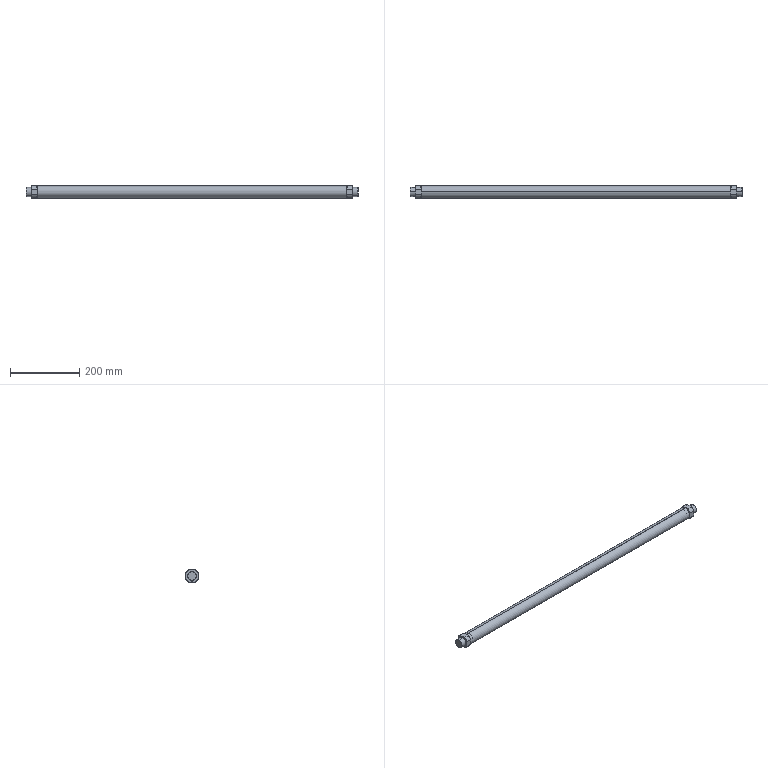Component | SolidWorks | RMS32X800_0-1_RMS32X800(0)-fcv-1 | 1 solid | 79 faces | volume 195434 mm3 | cylinder 30 | plane 19 | spline 16 | cone 14 | commonest cylinder face diameters 39.5 x8 5 x4 26 x4 10 x4 17 x4 32 x4 35 x2